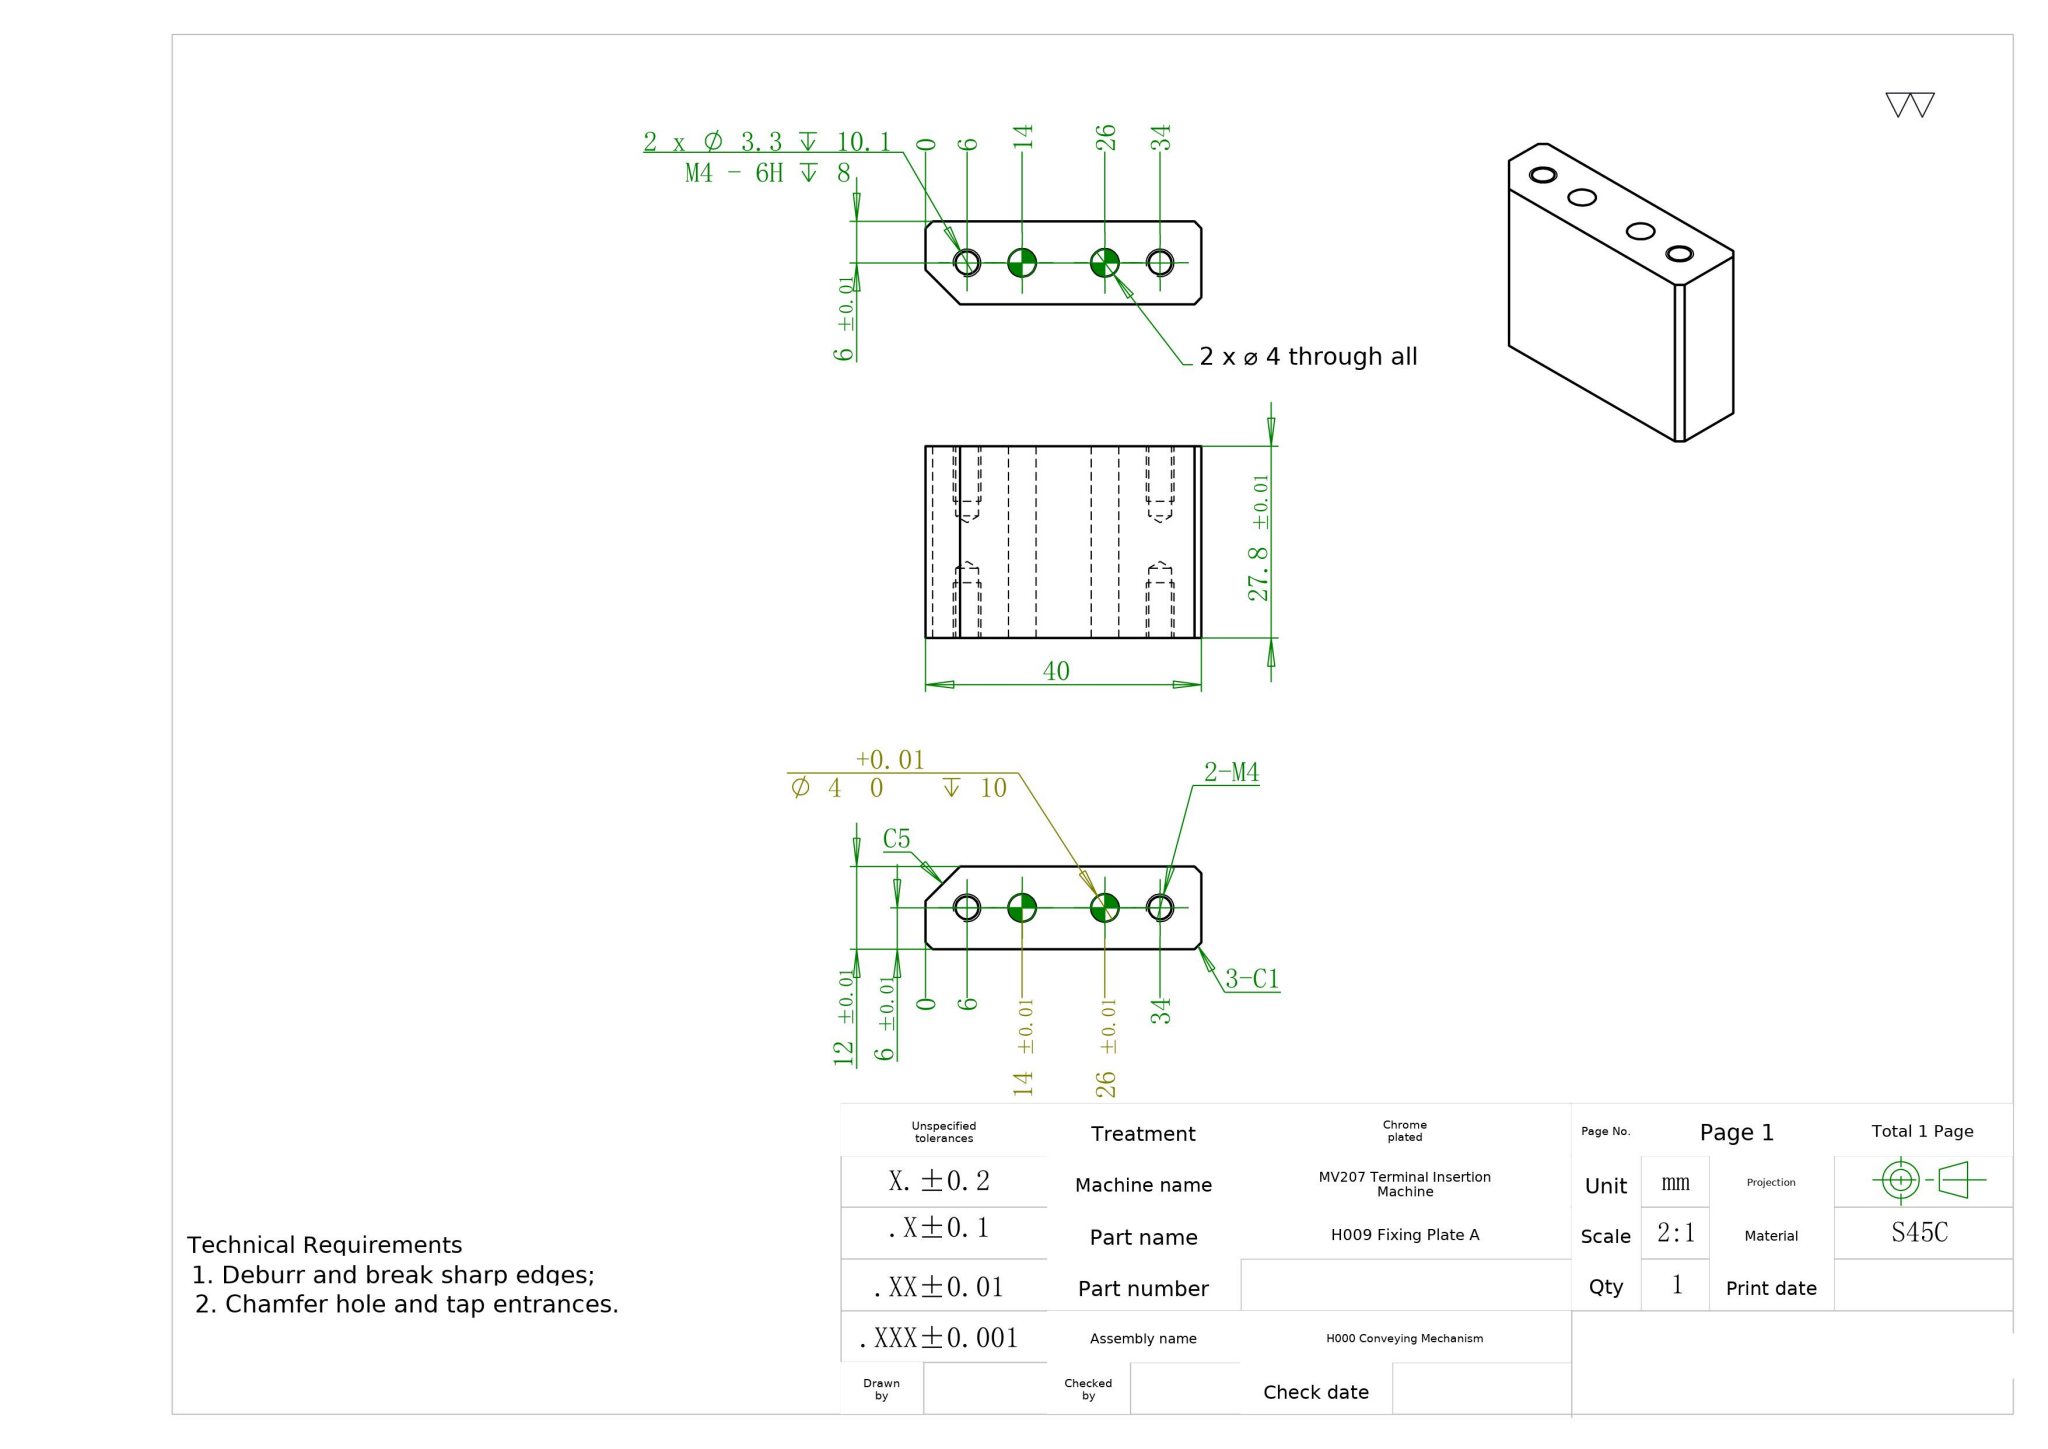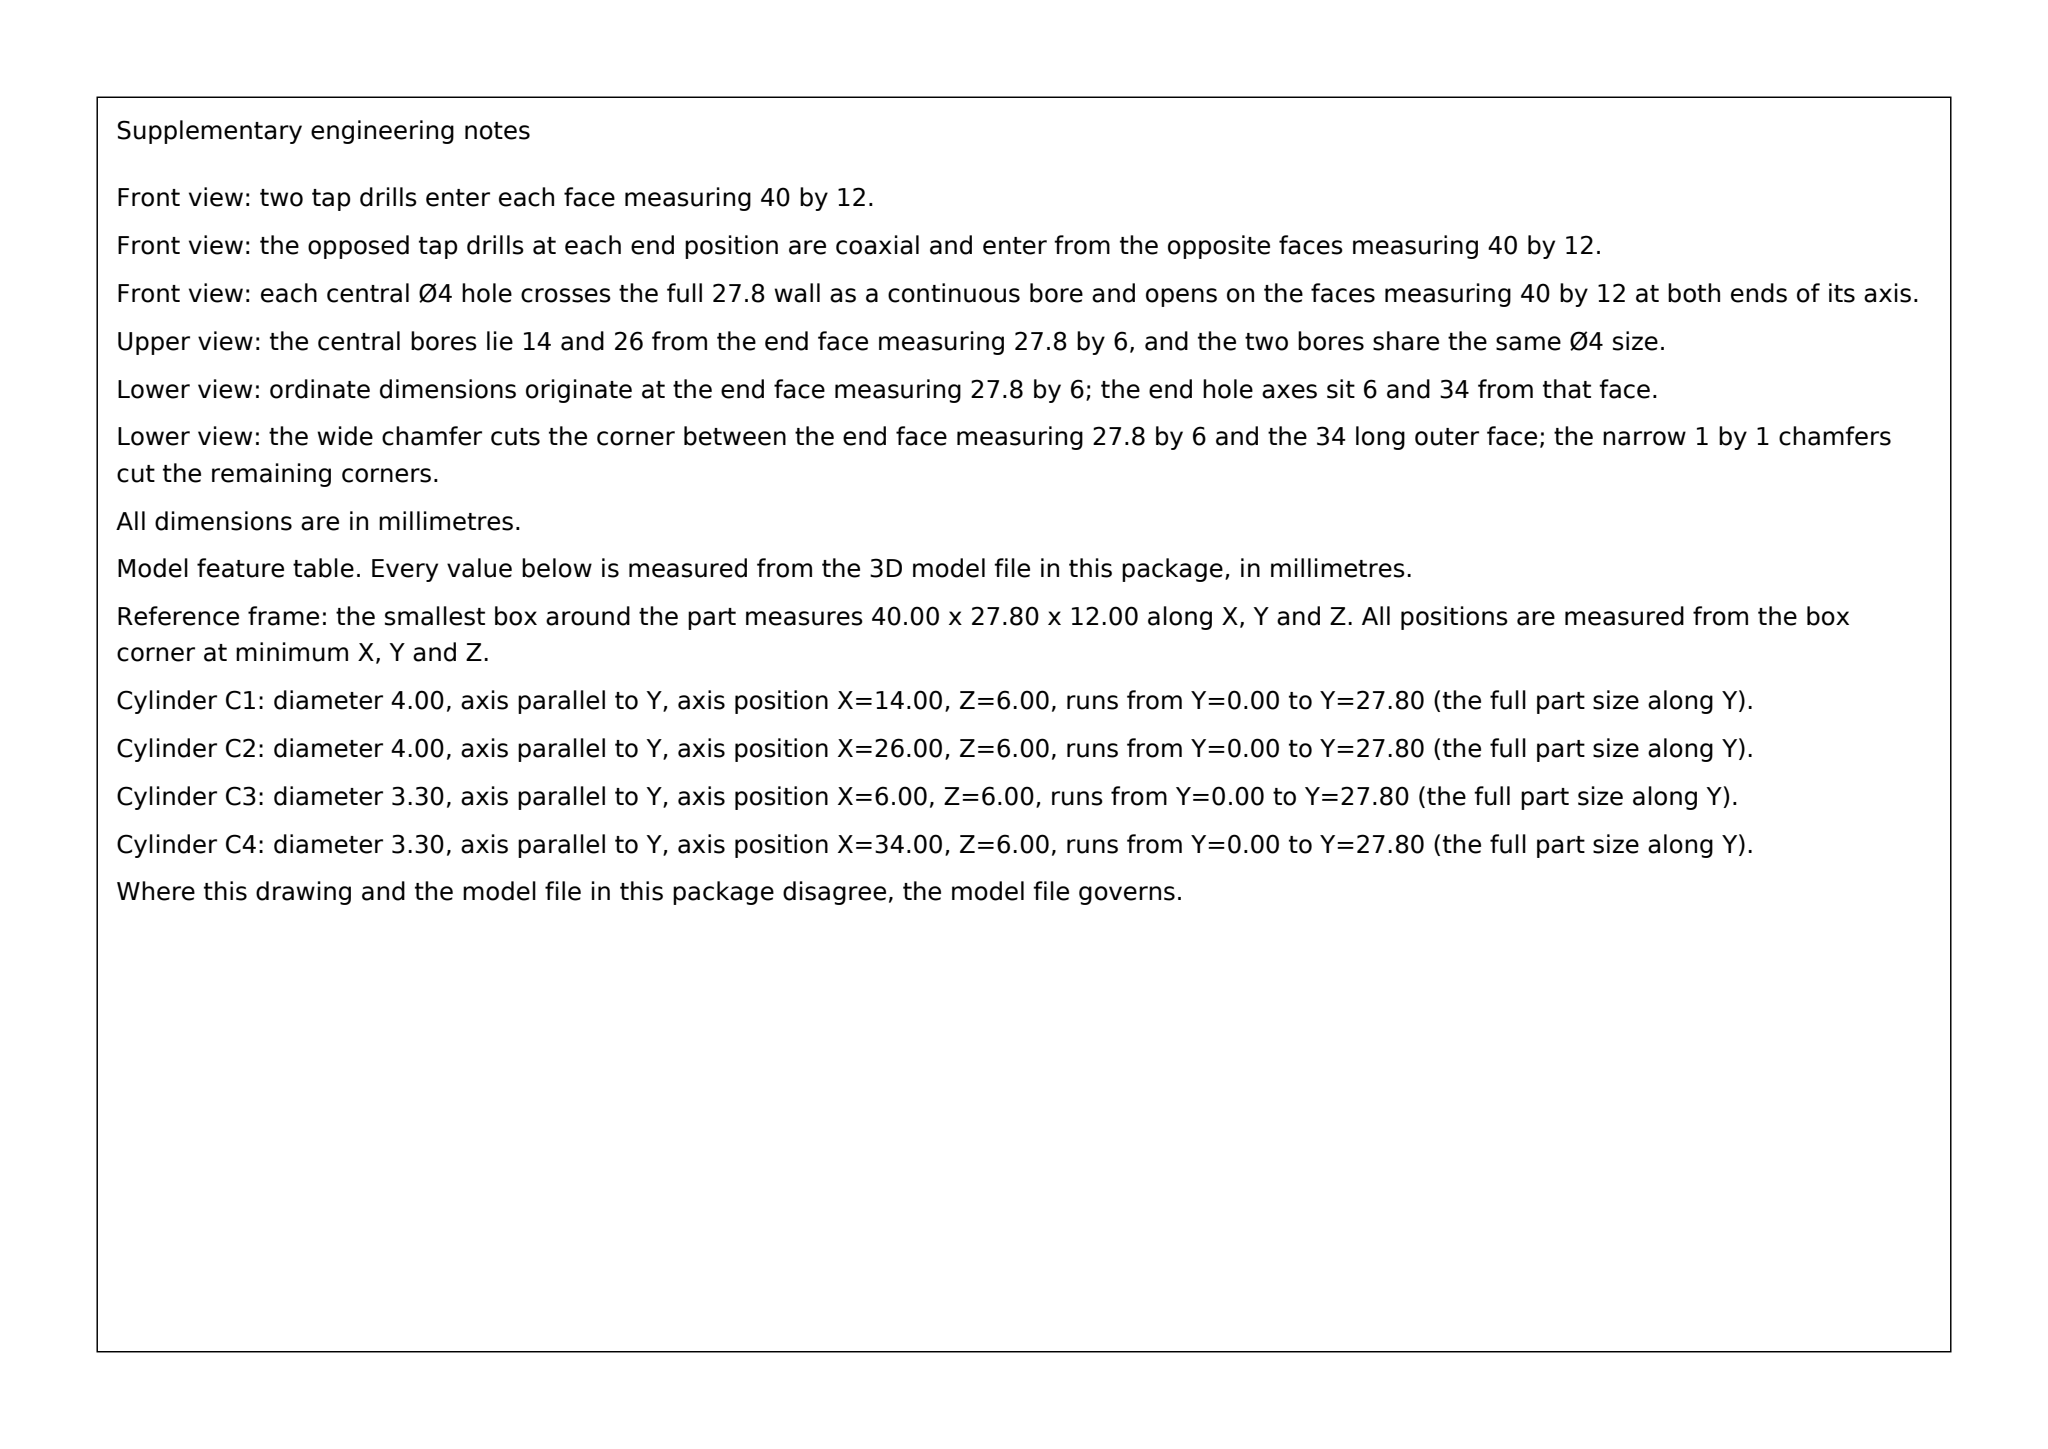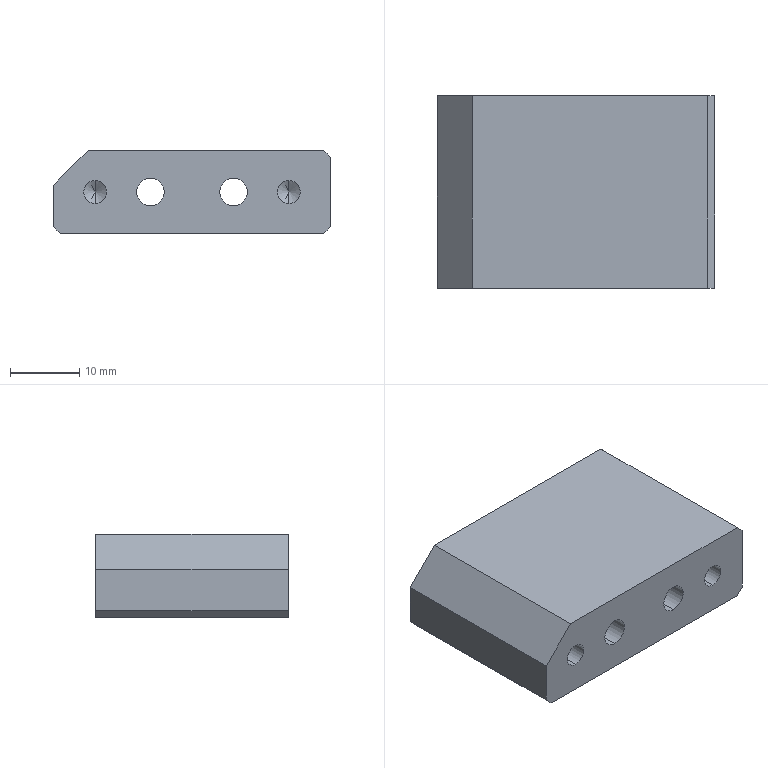Part | SolidWorks | mm | material S45C | 1 solid | 30 faces | box 40 x 27.8 x 12 mm | volume 11899 mm3 | cylinder 12 | plane 10 | cone 8 | commonest cylinder face diameters 3.3 x8 4 x4
Drawing notes:
2X Ø4 +0.01/0 THRU ALL = 27.8 DEEP (DISREGARD DP 10) | from the solid: Ø4 cylinders, axis Y, length 27.8 = full bbox Y (27.8) at x=14 & 26, z=6
TAPS: Ø3.3 DP 10.1 / M4-6H DP 8 FROM NEAREST 40X12 FACE | from the solid: Ø3.3 L=10.1 cyls (4 faces) + 8 cone faces @118°/Ø3.3 = 4 drill points, blind in 27.8 thk
4X M4-6H: 2 FROM TOP FACE, 2 FROM BOTTOM FACE, AT X=6 & 34, Z=6 | from the solid: Ø3.3 entries at [6,null,6] and [34,null,6], 4 cyl faces + 8 cone faces = 2 blind holes per location
DELETE C5: NO CHAMFER IN MODEL, CORNERS SQUARE 40 X 27.8 | from the solid: axis_planes only: x=0,40; y=0,27.8; z=0,12; no chamfer faces, fillet_radii=[]
DELETE 3-C1: NO C1 EDGES; ALL EDGES SHARP (BREAK EDGES ONLY) | from the solid: 6 planar faces form plain prism; no additional planar/conic edge faces present
PART IS PLAIN PRISM 40 X 27.8 X 12, NO CHAMFERS OR FILLETS | from the solid: bbox_xyz 40.0 x 27.8 x 12.0; 6 axis_planes; cones only 118 deg drill points on Ø3.3
build123d program:
from build123d import *

# Parameters (mm, degrees)
SKETCH1_W                    = 40
SKETCH1_H                    = 27.8
BOSS_EXTRUDE1_DEPTH          = 19.5
M4_TAPPED_HOLE2_D            = 3.3
M4_TAPPED_HOLE2_DEPTH        = 10.1
M4_TAPPED_HOLE2_TIP          = 0.9914
M4_TAPPED_HOLE1_D            = 3.3
M4_TAPPED_HOLE1_DEPTH        = 10.1
M4_TAPPED_HOLE1_TIP          = 0.9914
CHAMFER1_SIZE                = 5
F_4_0_4_DIAMETER_HOLE1_D     = 4
F_4_0_4_DIAMETER_HOLE2_D     = 4
F_4_0_4_DIAMETER_HOLE2_DEPTH = 10
F_4_0_4_DIAMETER_HOLE2_TIP   = 1.202
SKETCH15_W                   = 7.5
SKETCH15_H                   = 1.2
CUT_EXTRUDE1_DEPTH           = 47.62
SKETCH16_W                   = 40
SKETCH16_H                   = 25.4
CUT_EXTRUDE2_DEPTH           = 7.5
CHAMFER2_SIZE                = 1


with BuildPart() as part:
    # Sketch1 → Boss-Extrude1 (new body)
    with BuildSketch(Plane.XY):
        Rectangle(SKETCH1_W, SKETCH1_H)
    extrude(amount=BOSS_EXTRUDE1_DEPTH)

    # M4 Tapped Hole2
    with Locations(Plane(origin=(0, 13.9, 0), x_dir=(1, 0, 0), z_dir=(0, 1, 0))):
        with Locations((-14, -13.5), (14, -13.5)):
            Hole(M4_TAPPED_HOLE2_D / 2, depth=M4_TAPPED_HOLE2_DEPTH)
            with Locations((0, 0, -(M4_TAPPED_HOLE2_DEPTH + M4_TAPPED_HOLE2_TIP / 2))):  # 118° drill point
                Cone(0, M4_TAPPED_HOLE2_D / 2, M4_TAPPED_HOLE2_TIP, mode=Mode.SUBTRACT)

    # M4 Tapped Hole1
    with Locations(Plane(origin=(0, -13.9, 0), x_dir=(-1, 0, 0), z_dir=(0, -1, 0))):
        with Locations((14, -13.5), (-14, -13.5)):
            Hole(M4_TAPPED_HOLE1_D / 2, depth=M4_TAPPED_HOLE1_DEPTH)
            with Locations((0, 0, -(M4_TAPPED_HOLE1_DEPTH + M4_TAPPED_HOLE1_TIP / 2))):  # 118° drill point
                Cone(0, M4_TAPPED_HOLE1_D / 2, M4_TAPPED_HOLE1_TIP, mode=Mode.SUBTRACT)

    # Chamfer1
    chamfer1_edges = [part.edges().sort_by_distance(p)[0] for p in [
        (-20, 0, 19.5),
    ]]
    chamfer(chamfer1_edges, length=CHAMFER1_SIZE)

    # 4.0 _4_ Diameter Hole1 (through all)
    with Locations(Plane(origin=(0, 13.9, 0), x_dir=(1, 0, 0), z_dir=(0, 1, 0))):
        with Locations((-6, -13.5), (6, -13.5)):
            Hole(F_4_0_4_DIAMETER_HOLE1_D / 2)

    # 4.0 _4_ Diameter Hole2
    with Locations(Plane(origin=(0, -13.9, 0), x_dir=(-1, 0, 0), z_dir=(0, -1, 0))):
        with Locations((6, -13.5), (-6, -13.5)):
            Hole(F_4_0_4_DIAMETER_HOLE2_D / 2, depth=F_4_0_4_DIAMETER_HOLE2_DEPTH)
            with Locations((0, 0, -(F_4_0_4_DIAMETER_HOLE2_DEPTH + F_4_0_4_DIAMETER_HOLE2_TIP / 2))):  # 118° drill point
                Cone(0, F_4_0_4_DIAMETER_HOLE2_D / 2, F_4_0_4_DIAMETER_HOLE2_TIP, mode=Mode.SUBTRACT)

    # Sketch15 → Cut-Extrude1 (cut, through all)
    with BuildSketch(Plane(origin=(20, 0, 0), x_dir=(0, 0, -1), z_dir=(1, 0, 0))):
        with Locations((-3.75, -13.3)):
            Rectangle(SKETCH15_W, SKETCH15_H)
        with Locations((-3.75, 13.3)):
            Rectangle(SKETCH15_W, SKETCH15_H)
    extrude(amount=-CUT_EXTRUDE1_DEPTH, mode=Mode.SUBTRACT)

    # Sketch16 → Cut-Extrude2 (cut)
    with BuildSketch(Plane(origin=(0, 0, 0), x_dir=(-1, 0, 0), z_dir=(0, 0, -1))):
        Rectangle(SKETCH16_W, SKETCH16_H)
    extrude(amount=-CUT_EXTRUDE2_DEPTH, mode=Mode.SUBTRACT)

    # Chamfer2
    chamfer2_edges = [part.edges().sort_by_distance(p)[0] for p in [
        (20, 0, 19.5),
        (-20, 0, 7.5),
        (20, 0, 7.5),
    ]]
    chamfer(chamfer2_edges, length=CHAMFER2_SIZE)


solid = part.part
STEP:
#1=CARTESIAN_POINT('',(-6.,-13.9,11.5));
#2=VERTEX_POINT('',#1);
#3=CARTESIAN_POINT('',(-6.,-13.9,15.5));
#4=VERTEX_POINT('',#3);
#5=CARTESIAN_POINT('',(-6.,-13.9,13.5));
#6=DIRECTION('',(0.,1.,0.));
#7=DIRECTION('',(0.,0.,1.));
#8=AXIS2_PLACEMENT_3D('',#5,#6,#7);
#9=CIRCLE('',#8,2.);
#10=EDGE_CURVE('',#2,#4,#9,.T.);
#11=ORIENTED_EDGE('',*,*,#10,.F.);
#12=CARTESIAN_POINT('',(-6.,13.9,11.5));
#13=VERTEX_POINT('',#12);
#14=CARTESIAN_POINT('',(-6.,13.9,11.5));
#15=DIRECTION('',(0.,1.,0.));
#16=VECTOR('',#15,1000.);
#17=LINE('',#14,#16);
#18=EDGE_CURVE('',#2,#13,#17,.T.);
#19=ORIENTED_EDGE('',*,*,#18,.T.);
#20=CARTESIAN_POINT('',(-6.,13.9,15.5));
#21=VERTEX_POINT('',#20);
#22=CARTESIAN_POINT('',(-6.,13.9,13.5));
#23=DIRECTION('',(0.,1.,0.));
#24=DIRECTION('',(0.,0.,1.));
#25=AXIS2_PLACEMENT_3D('',#22,#23,#24);
#26=CIRCLE('',#25,2.);
#27=EDGE_CURVE('',#13,#21,#26,.T.);
#28=ORIENTED_EDGE('',*,*,#27,.T.);
#29=CARTESIAN_POINT('',(-6.,13.9,15.5));
#30=DIRECTION('',(0.,1.,0.));
#31=VECTOR('',#30,1000.);
#32=LINE('',#29,#31);
#33=EDGE_CURVE('',#4,#21,#32,.T.);
#34=ORIENTED_EDGE('',*,*,#33,.F.);
#35=EDGE_LOOP('',(#11,#19,#28,#34));
#36=FACE_OUTER_BOUND('',#35,.T.);
#37=CARTESIAN_POINT('',(-6.,13.9,13.5));
#38=DIRECTION('',(0.,1.,0.));
#39=DIRECTION('',(0.,0.,1.));
#40=AXIS2_PLACEMENT_3D('',#37,#38,#39);
#41=CYLINDRICAL_SURFACE('',#40,2.);
#42=ADVANCED_FACE('',(#36),#41,.F.);
#43=CARTESIAN_POINT('',(6.,-13.9,11.5));
#44=VERTEX_POINT('',#43);
#45=CARTESIAN_POINT('',(6.,-13.9,15.5));
#46=VERTEX_POINT('',#45);
#47=CARTESIAN_POINT('',(6.,-13.9,13.5));
#48=DIRECTION('',(0.,1.,0.));
#49=DIRECTION('',(0.,0.,1.));
#50=AXIS2_PLACEMENT_3D('',#47,#48,#49);
#51=CIRCLE('',#50,2.);
#52=EDGE_CURVE('',#44,#46,#51,.T.);
#53=ORIENTED_EDGE('',*,*,#52,.F.);
#54=CARTESIAN_POINT('',(6.,13.9,11.5));
#55=VERTEX_POINT('',#54);
#56=CARTESIAN_POINT('',(6.,13.9,11.5));
#57=DIRECTION('',(0.,1.,0.));
#58=VECTOR('',#57,1000.);
#59=LINE('',#56,#58);
#60=EDGE_CURVE('',#44,#55,#59,.T.);
#61=ORIENTED_EDGE('',*,*,#60,.T.);
#62=CARTESIAN_POINT('',(6.,13.9,15.5));
#63=VERTEX_POINT('',#62);
#64=CARTESIAN_POINT('',(6.,13.9,13.5));
#65=DIRECTION('',(0.,1.,0.));
#66=DIRECTION('',(0.,0.,1.));
#67=AXIS2_PLACEMENT_3D('',#64,#65,#66);
#68=CIRCLE('',#67,2.);
#69=EDGE_CURVE('',#55,#63,#68,.T.);
#70=ORIENTED_EDGE('',*,*,#69,.T.);
#71=CARTESIAN_POINT('',(6.,13.9,15.5));
#72=DIRECTION('',(0.,1.,0.));
#73=VECTOR('',#72,1000.);
#74=LINE('',#71,#73);
#75=EDGE_CURVE('',#46,#63,#74,.T.);
#76=ORIENTED_EDGE('',*,*,#75,.F.);
#77=EDGE_LOOP('',(#53,#61,#70,#76));
#78=FACE_OUTER_BOUND('',#77,.T.);
#79=CARTESIAN_POINT('',(6.,13.9,13.5));
#80=DIRECTION('',(0.,1.,0.));
#81=DIRECTION('',(0.,0.,1.));
#82=AXIS2_PLACEMENT_3D('',#79,#80,#81);
#83=CYLINDRICAL_SURFACE('',#82,2.);
#84=ADVANCED_FACE('',(#78),#83,.F.);
#85=CARTESIAN_POINT('',(-14.,-3.8,15.15));
#86=VERTEX_POINT('',#85);
#87=CARTESIAN_POINT('',(-14.,-3.8,11.85));
#88=VERTEX_POINT('',#87);
#89=CARTESIAN_POINT('',(-14.,-3.8,13.5));
#90=DIRECTION('',(0.,-1.,0.));
#91=DIRECTION('',(0.,0.,-1.));
#92=AXIS2_PLACEMENT_3D('',#89,#90,#91);
#93=CIRCLE('',#92,1.65);
#94=EDGE_CURVE('',#86,#88,#93,.T.);
#95=ORIENTED_EDGE('',*,*,#94,.F.);
#96=CARTESIAN_POINT('',(-14.,-13.9,15.15));
#97=VERTEX_POINT('',#96);
#98=CARTESIAN_POINT('',(-14.,-13.9,15.15));
#99=DIRECTION('',(0.,-1.,0.));
#100=VECTOR('',#99,1000.);
#101=LINE('',#98,#100);
#102=EDGE_CURVE('',#86,#97,#101,.T.);
#103=ORIENTED_EDGE('',*,*,#102,.T.);
#104=CARTESIAN_POINT('',(-14.,-13.9,11.85));
#105=VERTEX_POINT('',#104);
#106=CARTESIAN_POINT('',(-14.,-13.9,13.5));
#107=DIRECTION('',(0.,-1.,0.));
#108=DIRECTION('',(0.,0.,-1.));
#109=AXIS2_PLACEMENT_3D('',#106,#107,#108);
#110=CIRCLE('',#109,1.65);
#111=EDGE_CURVE('',#97,#105,#110,.T.);
#112=ORIENTED_EDGE('',*,*,#111,.T.);
#113=CARTESIAN_POINT('',(-14.,-13.9,11.85));
#114=DIRECTION('',(0.,-1.,0.));
#115=VECTOR('',#114,1000.);
#116=LINE('',#113,#115);
#117=EDGE_CURVE('',#88,#105,#116,.T.);
#118=ORIENTED_EDGE('',*,*,#117,.F.);
#119=EDGE_LOOP('',(#95,#103,#112,#118));
#120=FACE_OUTER_BOUND('',#119,.T.);
#121=CARTESIAN_POINT('',(-14.,-13.9,13.5));
#122=DIRECTION('',(0.,-1.,0.));
#123=DIRECTION('',(0.,0.,-1.));
#124=AXIS2_PLACEMENT_3D('',#121,#122,#123);
#125=CYLINDRICAL_SURFACE('',#124,1.65);
#126=ADVANCED_FACE('',(#120),#125,.F.);
#127=CARTESIAN_POINT('',(-14.,-2.809,13.5));
#128=VERTEX_POINT('',#127);
#129=CARTESIAN_POINT('',(-14.,-3.8,11.85));
#130=DIRECTION('',(0.,-0.515,-0.8572));
#131=VECTOR('',#130,1000.);
#132=LINE('',#129,#131);
#133=EDGE_CURVE('',#128,#88,#132,.T.);
#134=ORIENTED_EDGE('',*,*,#133,.F.);
#135=CARTESIAN_POINT('',(-14.,-3.8,15.15));
#136=DIRECTION('',(0.,-0.515,0.8572));
#137=VECTOR('',#136,1000.);
#138=LINE('',#135,#137);
#139=EDGE_CURVE('',#128,#86,#138,.T.);
#140=ORIENTED_EDGE('',*,*,#139,.T.);
#141=ORIENTED_EDGE('',*,*,#94,.T.);
#142=EDGE_LOOP('',(#134,#140,#141));
#143=FACE_OUTER_BOUND('',#142,.T.);
#144=CARTESIAN_POINT('',(-14.,-3.8,13.5));
#145=DIRECTION('',(0.,-1.,0.));
#146=DIRECTION('',(0.,0.,-1.));
#147=AXIS2_PLACEMENT_3D('',#144,#145,#146);
#148=CONICAL_SURFACE('',#147,1.65,1.03);
#149=ADVANCED_FACE('',(#143),#148,.F.);
#150=CARTESIAN_POINT('',(14.,-3.8,15.15));
#151=VERTEX_POINT('',#150);
#152=CARTESIAN_POINT('',(14.,-3.8,11.85));
#153=VERTEX_POINT('',#152);
#154=CARTESIAN_POINT('',(14.,-3.8,13.5));
#155=DIRECTION('',(0.,-1.,0.));
#156=DIRECTION('',(0.,0.,-1.));
#157=AXIS2_PLACEMENT_3D('',#154,#155,#156);
#158=CIRCLE('',#157,1.65);
#159=EDGE_CURVE('',#151,#153,#158,.T.);
#160=ORIENTED_EDGE('',*,*,#159,.F.);
#161=CARTESIAN_POINT('',(14.,-13.9,15.15));
#162=VERTEX_POINT('',#161);
#163=CARTESIAN_POINT('',(14.,-13.9,15.15));
#164=DIRECTION('',(0.,-1.,0.));
#165=VECTOR('',#164,1000.);
#166=LINE('',#163,#165);
#167=EDGE_CURVE('',#151,#162,#166,.T.);
#168=ORIENTED_EDGE('',*,*,#167,.T.);
#169=CARTESIAN_POINT('',(14.,-13.9,11.85));
#170=VERTEX_POINT('',#169);
#171=CARTESIAN_POINT('',(14.,-13.9,13.5));
#172=DIRECTION('',(0.,-1.,0.));
#173=DIRECTION('',(0.,0.,-1.));
#174=AXIS2_PLACEMENT_3D('',#171,#172,#173);
#175=CIRCLE('',#174,1.65);
#176=EDGE_CURVE('',#162,#170,#175,.T.);
#177=ORIENTED_EDGE('',*,*,#176,.T.);
#178=CARTESIAN_POINT('',(14.,-13.9,11.85));
#179=DIRECTION('',(0.,-1.,0.));
#180=VECTOR('',#179,1000.);
#181=LINE('',#178,#180);
#182=EDGE_CURVE('',#153,#170,#181,.T.);
#183=ORIENTED_EDGE('',*,*,#182,.F.);
#184=EDGE_LOOP('',(#160,#168,#177,#183));
#185=FACE_OUTER_BOUND('',#184,.T.);
#186=CARTESIAN_POINT('',(14.,-13.9,13.5));
#187=DIRECTION('',(0.,-1.,0.));
#188=DIRECTION('',(0.,0.,-1.));
#189=AXIS2_PLACEMENT_3D('',#186,#187,#188);
#190=CYLINDRICAL_SURFACE('',#189,1.65);
#191=ADVANCED_FACE('',(#185),#190,.F.);
#192=CARTESIAN_POINT('',(14.,-2.809,13.5));
#193=VERTEX_POINT('',#192);
#194=CARTESIAN_POINT('',(14.,-3.8,11.85));
#195=DIRECTION('',(0.,-0.515,-0.8572));
#196=VECTOR('',#195,1000.);
#197=LINE('',#194,#196);
#198=EDGE_CURVE('',#193,#153,#197,.T.);
#199=ORIENTED_EDGE('',*,*,#198,.F.);
#200=CARTESIAN_POINT('',(14.,-3.8,15.15));
#201=DIRECTION('',(0.,-0.515,0.8572));
#202=VECTOR('',#201,1000.);
#203=LINE('',#200,#202);
#204=EDGE_CURVE('',#193,#151,#203,.T.);
#205=ORIENTED_EDGE('',*,*,#204,.T.);
#206=ORIENTED_EDGE('',*,*,#159,.T.);
#207=EDGE_LOOP('',(#199,#205,#206));
#208=FACE_OUTER_BOUND('',#207,.T.);
#209=CARTESIAN_POINT('',(14.,-3.8,13.5));
#210=DIRECTION('',(0.,-1.,0.));
#211=DIRECTION('',(0.,0.,-1.));
#212=AXIS2_PLACEMENT_3D('',#209,#210,#211);
#213=CONICAL_SURFACE('',#212,1.65,1.03);
#214=ADVANCED_FACE('',(#208),#213,.F.);
#215=CARTESIAN_POINT('',(-14.,3.8,11.85));
#216=VERTEX_POINT('',#215);
#217=CARTESIAN_POINT('',(-14.,3.8,15.15));
#218=VERTEX_POINT('',#217);
#219=CARTESIAN_POINT('',(-14.,3.8,13.5));
#220=DIRECTION('',(0.,1.,0.));
#221=DIRECTION('',(0.,0.,1.));
#222=AXIS2_PLACEMENT_3D('',#219,#220,#221);
#223=CIRCLE('',#222,1.65);
#224=EDGE_CURVE('',#216,#218,#223,.T.);
#225=ORIENTED_EDGE('',*,*,#224,.F.);
#226=CARTESIAN_POINT('',(-14.,13.9,11.85));
#227=VERTEX_POINT('',#226);
#228=CARTESIAN_POINT('',(-14.,13.9,11.85));
#229=DIRECTION('',(0.,1.,0.));
#230=VECTOR('',#229,1000.);
#231=LINE('',#228,#230);
#232=EDGE_CURVE('',#216,#227,#231,.T.);
#233=ORIENTED_EDGE('',*,*,#232,.T.);
#234=CARTESIAN_POINT('',(-14.,13.9,15.15));
#235=VERTEX_POINT('',#234);
#236=CARTESIAN_POINT('',(-14.,13.9,13.5));
#237=DIRECTION('',(0.,1.,0.));
#238=DIRECTION('',(0.,0.,1.));
#239=AXIS2_PLACEMENT_3D('',#236,#237,#238);
#240=CIRCLE('',#239,1.65);
#241=EDGE_CURVE('',#227,#235,#240,.T.);
#242=ORIENTED_EDGE('',*,*,#241,.T.);
#243=CARTESIAN_POINT('',(-14.,13.9,15.15));
#244=DIRECTION('',(0.,1.,0.));
#245=VECTOR('',#244,1000.);
#246=LINE('',#243,#245);
#247=EDGE_CURVE('',#218,#235,#246,.T.);
#248=ORIENTED_EDGE('',*,*,#247,.F.);
#249=EDGE_LOOP('',(#225,#233,#242,#248));
#250=FACE_OUTER_BOUND('',#249,.T.);
#251=CARTESIAN_POINT('',(-14.,13.9,13.5));
#252=DIRECTION('',(0.,1.,0.));
#253=DIRECTION('',(0.,0.,1.));
#254=AXIS2_PLACEMENT_3D('',#251,#252,#253);
#255=CYLINDRICAL_SURFACE('',#254,1.65);
#256=ADVANCED_FACE('',(#250),#255,.F.);
#257=CARTESIAN_POINT('',(-14.,2.809,13.5));
#258=VERTEX_POINT('',#257);
#259=CARTESIAN_POINT('',(-14.,3.8,15.15));
#260=DIRECTION('',(0.,0.515,0.8572));
#261=VECTOR('',#260,1000.);
#262=LINE('',#259,#261);
#263=EDGE_CURVE('',#258,#218,#262,.T.);
#264=ORIENTED_EDGE('',*,*,#263,.F.);
#265=CARTESIAN_POINT('',(-14.,3.8,11.85));
#266=DIRECTION('',(0.,0.515,-0.8572));
#267=VECTOR('',#266,1000.);
#268=LINE('',#265,#267);
#269=EDGE_CURVE('',#258,#216,#268,.T.);
#270=ORIENTED_EDGE('',*,*,#269,.T.);
#271=ORIENTED_EDGE('',*,*,#224,.T.);
#272=EDGE_LOOP('',(#264,#270,#271));
#273=FACE_OUTER_BOUND('',#272,.T.);
#274=CARTESIAN_POINT('',(-14.,3.8,13.5));
#275=DIRECTION('',(0.,1.,0.));
#276=DIRECTION('',(0.,0.,1.));
#277=AXIS2_PLACEMENT_3D('',#274,#275,#276);
#278=CONICAL_SURFACE('',#277,1.65,1.03);
#279=ADVANCED_FACE('',(#273),#278,.F.);
#280=CARTESIAN_POINT('',(14.,3.8,11.85));
#281=VERTEX_POINT('',#280);
#282=CARTESIAN_POINT('',(14.,3.8,15.15));
#283=VERTEX_POINT('',#282);
#284=CARTESIAN_POINT('',(14.,3.8,13.5));
#285=DIRECTION('',(0.,1.,0.));
#286=DIRECTION('',(0.,0.,1.));
#287=AXIS2_PLACEMENT_3D('',#284,#285,#286);
#288=CIRCLE('',#287,1.65);
#289=EDGE_CURVE('',#281,#283,#288,.T.);
#290=ORIENTED_EDGE('',*,*,#289,.F.);
#291=CARTESIAN_POINT('',(14.,13.9,11.85));
#292=VERTEX_POINT('',#291);
#293=CARTESIAN_POINT('',(14.,13.9,11.85));
#294=DIRECTION('',(0.,1.,0.));
#295=VECTOR('',#294,1000.);
#296=LINE('',#293,#295);
#297=EDGE_CURVE('',#281,#292,#296,.T.);
#298=ORIENTED_EDGE('',*,*,#297,.T.);
#299=CARTESIAN_POINT('',(14.,13.9,15.15));
#300=VERTEX_POINT('',#299);
#301=CARTESIAN_POINT('',(14.,13.9,13.5));
#302=DIRECTION('',(0.,1.,0.));
#303=DIRECTION('',(0.,0.,1.));
#304=AXIS2_PLACEMENT_3D('',#301,#302,#303);
#305=CIRCLE('',#304,1.65);
#306=EDGE_CURVE('',#292,#300,#305,.T.);
#307=ORIENTED_EDGE('',*,*,#306,.T.);
#308=CARTESIAN_POINT('',(14.,13.9,15.15));
#309=DIRECTION('',(0.,1.,0.));
#310=VECTOR('',#309,1000.);
#311=LINE('',#308,#310);
#312=EDGE_CURVE('',#283,#300,#311,.T.);
#313=ORIENTED_EDGE('',*,*,#312,.F.);
#314=EDGE_LOOP('',(#290,#298,#307,#313));
#315=FACE_OUTER_BOUND('',#314,.T.);
#316=CARTESIAN_POINT('',(14.,13.9,13.5));
#317=DIRECTION('',(0.,1.,0.));
#318=DIRECTION('',(0.,0.,1.));
#319=AXIS2_PLACEMENT_3D('',#316,#317,#318);
#320=CYLINDRICAL_SURFACE('',#319,1.65);
#321=ADVANCED_FACE('',(#315),#320,.F.);
#322=CARTESIAN_POINT('',(14.,2.809,13.5));
#323=VERTEX_POINT('',#322);
#324=CARTESIAN_POINT('',(14.,3.8,15.15));
#325=DIRECTION('',(0.,0.515,0.8572));
#326=VECTOR('',#325,1000.);
#327=LINE('',#324,#326);
#328=EDGE_CURVE('',#323,#283,#327,.T.);
#329=ORIENTED_EDGE('',*,*,#328,.F.);
#330=CARTESIAN_POINT('',(14.,3.8,11.85));
#331=DIRECTION('',(0.,0.515,-0.8572));
#332=VECTOR('',#331,1000.);
#333=LINE('',#330,#332);
#334=EDGE_CURVE('',#323,#281,#333,.T.);
#335=ORIENTED_EDGE('',*,*,#334,.T.);
#336=ORIENTED_EDGE('',*,*,#289,.T.);
#337=EDGE_LOOP('',(#329,#335,#336));
#338=FACE_OUTER_BOUND('',#337,.T.);
#339=CARTESIAN_POINT('',(14.,3.8,13.5));
#340=DIRECTION('',(0.,1.,0.));
#341=DIRECTION('',(0.,0.,1.));
#342=AXIS2_PLACEMENT_3D('',#339,#340,#341);
#343=CONICAL_SURFACE('',#342,1.65,1.03);
#344=ADVANCED_FACE('',(#338),#343,.F.);
#345=CARTESIAN_POINT('',(20.,13.9,18.5));
#346=VERTEX_POINT('',#345);
#347=CARTESIAN_POINT('',(20.,13.9,8.5));
#348=VERTEX_POINT('',#347);
#349=CARTESIAN_POINT('',(20.,13.9,19.5));
#350=DIRECTION('',(0.,0.,-1.));
#351=VECTOR('',#350,1000.);
#352=LINE('',#349,#351);
#353=EDGE_CURVE('',#346,#348,#352,.T.);
#354=ORIENTED_EDGE('',*,*,#353,.F.);
#355=CARTESIAN_POINT('',(20.,-13.9,18.5));
#356=VERTEX_POINT('',#355);
#357=CARTESIAN_POINT('',(20.,-13.9,18.5));
#358=DIRECTION('',(0.,-1.,0.));
#359=VECTOR('',#358,1000.);
#360=LINE('',#357,#359);
#361=EDGE_CURVE('',#346,#356,#360,.T.);
#362=ORIENTED_EDGE('',*,*,#361,.T.);
#363=CARTESIAN_POINT('',(20.,-13.9,8.5));
#364=VERTEX_POINT('',#363);
#365=CARTESIAN_POINT('',(20.,-13.9,19.5));
#366=DIRECTION('',(0.,0.,-1.));
#367=VECTOR('',#366,1000.);
#368=LINE('',#365,#367);
#369=EDGE_CURVE('',#356,#364,#368,.T.);
#370=ORIENTED_EDGE('',*,*,#369,.T.);
#371=CARTESIAN_POINT('',(20.,13.9,8.5));
#372=DIRECTION('',(0.,1.,0.));
#373=VECTOR('',#372,1000.);
#374=LINE('',#371,#373);
#375=EDGE_CURVE('',#364,#348,#374,.T.);
#376=ORIENTED_EDGE('',*,*,#375,.T.);
#377=EDGE_LOOP('',(#354,#362,#370,#376));
#378=FACE_OUTER_BOUND('',#377,.T.);
#379=CARTESIAN_POINT('',(20.,13.9,19.5));
#380=DIRECTION('',(-1.,0.,0.));
#381=DIRECTION('',(0.,0.,1.));
#382=AXIS2_PLACEMENT_3D('',#379,#380,#381);
#383=PLANE('',#382);
#384=ADVANCED_FACE('',(#378),#383,.F.);
#385=CARTESIAN_POINT('',(-6.,13.9,13.5));
#386=DIRECTION('',(0.,1.,0.));
#387=DIRECTION('',(0.,0.,1.));
#388=AXIS2_PLACEMENT_3D('',#385,#386,#387);
#389=CIRCLE('',#388,2.);
#390=EDGE_CURVE('',#21,#13,#389,.T.);
#391=ORIENTED_EDGE('',*,*,#390,.F.);
#392=ORIENTED_EDGE('',*,*,#27,.F.);
#393=EDGE_LOOP('',(#391,#392));
#394=FACE_BOUND('',#393,.T.);
#395=CARTESIAN_POINT('',(6.,13.9,13.5));
#396=DIRECTION('',(0.,1.,0.));
#397=DIRECTION('',(0.,0.,1.));
#398=AXIS2_PLACEMENT_3D('',#395,#396,#397);
#399=CIRCLE('',#398,2.);
#400=EDGE_CURVE('',#63,#55,#399,.T.);
#401=ORIENTED_EDGE('',*,*,#400,.F.);
#402=ORIENTED_EDGE('',*,*,#69,.F.);
#403=EDGE_LOOP('',(#401,#402));
#404=FACE_BOUND('',#403,.T.);
#405=CARTESIAN_POINT('',(-14.,13.9,13.5));
#406=DIRECTION('',(0.,1.,0.));
#407=DIRECTION('',(0.,0.,1.));
#408=AXIS2_PLACEMENT_3D('',#405,#406,#407);
#409=CIRCLE('',#408,1.65);
#410=EDGE_CURVE('',#235,#227,#409,.T.);
#411=ORIENTED_EDGE('',*,*,#410,.F.);
#412=ORIENTED_EDGE('',*,*,#241,.F.);
#413=EDGE_LOOP('',(#411,#412));
#414=FACE_BOUND('',#413,.T.);
#415=CARTESIAN_POINT('',(14.,13.9,13.5));
#416=DIRECTION('',(0.,1.,0.));
#417=DIRECTION('',(0.,0.,1.));
#418=AXIS2_PLACEMENT_3D('',#415,#416,#417);
#419=CIRCLE('',#418,1.65);
#420=EDGE_CURVE('',#300,#292,#419,.T.);
#421=ORIENTED_EDGE('',*,*,#420,.F.);
#422=ORIENTED_EDGE('',*,*,#306,.F.);
#423=EDGE_LOOP('',(#421,#422));
#424=FACE_BOUND('',#423,.T.);
#425=CARTESIAN_POINT('',(19.,13.9,19.5));
#426=VERTEX_POINT('',#425);
#427=CARTESIAN_POINT('',(-15.,13.9,19.5));
#428=VERTEX_POINT('',#427);
#429=CARTESIAN_POINT('',(-20.,13.9,19.5));
#430=DIRECTION('',(-1.,0.,0.));
#431=VECTOR('',#430,1000.);
#432=LINE('',#429,#431);
#433=EDGE_CURVE('',#426,#428,#432,.T.);
#434=ORIENTED_EDGE('',*,*,#433,.F.);
#435=CARTESIAN_POINT('',(19.,13.9,19.5));
#436=DIRECTION('',(0.7071,0.,-0.7071));
#437=VECTOR('',#436,1000.);
#438=LINE('',#435,#437);
#439=EDGE_CURVE('',#426,#346,#438,.T.);
#440=ORIENTED_EDGE('',*,*,#439,.T.);
#441=ORIENTED_EDGE('',*,*,#353,.T.);
#442=CARTESIAN_POINT('',(19.,13.9,7.5));
#443=VERTEX_POINT('',#442);
#444=CARTESIAN_POINT('',(19.,13.9,7.5));
#445=DIRECTION('',(-0.7071,0.,-0.7071));
#446=VECTOR('',#445,1000.);
#447=LINE('',#444,#446);
#448=EDGE_CURVE('',#348,#443,#447,.T.);
#449=ORIENTED_EDGE('',*,*,#448,.T.);
#450=CARTESIAN_POINT('',(-19.,13.9,7.5));
#451=VERTEX_POINT('',#450);
#452=CARTESIAN_POINT('',(-20.,13.9,7.5));
#453=DIRECTION('',(1.,0.,0.));
#454=VECTOR('',#453,1000.);
#455=LINE('',#452,#454);
#456=EDGE_CURVE('',#451,#443,#455,.T.);
#457=ORIENTED_EDGE('',*,*,#456,.F.);
#458=CARTESIAN_POINT('',(-20.,13.9,8.5));
#459=VERTEX_POINT('',#458);
#460=CARTESIAN_POINT('',(-20.,13.9,8.5));
#461=DIRECTION('',(-0.7071,0.,0.7071));
#462=VECTOR('',#461,1000.);
#463=LINE('',#460,#462);
#464=EDGE_CURVE('',#451,#459,#463,.T.);
#465=ORIENTED_EDGE('',*,*,#464,.T.);
#466=CARTESIAN_POINT('',(-20.,13.9,14.5));
#467=VERTEX_POINT('',#466);
#468=CARTESIAN_POINT('',(-20.,13.9,19.5));
#469=DIRECTION('',(0.,0.,-1.));
#470=VECTOR('',#469,1000.);
#471=LINE('',#468,#470);
#472=EDGE_CURVE('',#467,#459,#471,.T.);
#473=ORIENTED_EDGE('',*,*,#472,.F.);
#474=CARTESIAN_POINT('',(-15.,13.9,19.5));
#475=DIRECTION('',(0.7071,0.,0.7071));
#476=VECTOR('',#475,1000.);
#477=LINE('',#474,#476);
#478=EDGE_CURVE('',#467,#428,#477,.T.);
#479=ORIENTED_EDGE('',*,*,#478,.T.);
#480=EDGE_LOOP('',(#434,#440,#441,#449,#457,#465,#473,#479));
#481=FACE_OUTER_BOUND('',#480,.T.);
#482=CARTESIAN_POINT('',(-20.,13.9,19.5));
#483=DIRECTION('',(0.,-1.,0.));
#484=DIRECTION('',(0.,0.,-1.));
#485=AXIS2_PLACEMENT_3D('',#482,#483,#484);
#486=PLANE('',#485);
#487=ADVANCED_FACE('',(#394,#404,#414,#424,#481),#486,.F.);
#488=ORIENTED_EDGE('',*,*,#472,.T.);
#489=CARTESIAN_POINT('',(-20.,-13.9,8.5));
#490=VERTEX_POINT('',#489);
#491=CARTESIAN_POINT('',(-20.,13.9,8.5));
#492=DIRECTION('',(0.,-1.,0.));
#493=VECTOR('',#492,1000.);
#494=LINE('',#491,#493);
#495=EDGE_CURVE('',#459,#490,#494,.T.);
#496=ORIENTED_EDGE('',*,*,#495,.T.);
#497=CARTESIAN_POINT('',(-20.,-13.9,14.5));
#498=VERTEX_POINT('',#497);
#499=CARTESIAN_POINT('',(-20.,-13.9,19.5));
#500=DIRECTION('',(0.,0.,-1.));
#501=VECTOR('',#500,1000.);
#502=LINE('',#499,#501);
#503=EDGE_CURVE('',#498,#490,#502,.T.);
#504=ORIENTED_EDGE('',*,*,#503,.F.);
#505=CARTESIAN_POINT('',(-20.,13.9,14.5));
#506=DIRECTION('',(0.,1.,0.));
#507=VECTOR('',#506,1000.);
#508=LINE('',#505,#507);
#509=EDGE_CURVE('',#498,#467,#508,.T.);
#510=ORIENTED_EDGE('',*,*,#509,.T.);
#511=EDGE_LOOP('',(#488,#496,#504,#510));
#512=FACE_OUTER_BOUND('',#511,.T.);
#513=CARTESIAN_POINT('',(-20.,13.9,19.5));
#514=DIRECTION('',(1.,0.,0.));
#515=DIRECTION('',(0.,0.,-1.));
#516=AXIS2_PLACEMENT_3D('',#513,#514,#515);
#517=PLANE('',#516);
#518=ADVANCED_FACE('',(#512),#517,.F.);
#519=CARTESIAN_POINT('',(-6.,-13.9,13.5));
#520=DIRECTION('',(0.,1.,0.));
#521=DIRECTION('',(0.,0.,1.));
#522=AXIS2_PLACEMENT_3D('',#519,#520,#521);
#523=CIRCLE('',#522,2.);
#524=EDGE_CURVE('',#4,#2,#523,.T.);
#525=ORIENTED_EDGE('',*,*,#524,.T.);
#526=ORIENTED_EDGE('',*,*,#10,.T.);
#527=EDGE_LOOP('',(#525,#526));
#528=FACE_BOUND('',#527,.T.);
#529=CARTESIAN_POINT('',(6.,-13.9,13.5));
#530=DIRECTION('',(0.,1.,0.));
#531=DIRECTION('',(0.,0.,1.));
#532=AXIS2_PLACEMENT_3D('',#529,#530,#531);
#533=CIRCLE('',#532,2.);
#534=EDGE_CURVE('',#46,#44,#533,.T.);
#535=ORIENTED_EDGE('',*,*,#534,.T.);
#536=ORIENTED_EDGE('',*,*,#52,.T.);
#537=EDGE_LOOP('',(#535,#536));
#538=FACE_BOUND('',#537,.T.);
#539=CARTESIAN_POINT('',(-14.,-13.9,13.5));
#540=DIRECTION('',(0.,-1.,0.));
#541=DIRECTION('',(0.,0.,-1.));
#542=AXIS2_PLACEMENT_3D('',#539,#540,#541);
#543=CIRCLE('',#542,1.65);
#544=EDGE_CURVE('',#105,#97,#543,.T.);
#545=ORIENTED_EDGE('',*,*,#544,.F.);
#546=ORIENTED_EDGE('',*,*,#111,.F.);
#547=EDGE_LOOP('',(#545,#546));
#548=FACE_BOUND('',#547,.T.);
#549=CARTESIAN_POINT('',(14.,-13.9,13.5));
#550=DIRECTION('',(0.,-1.,0.));
#551=DIRECTION('',(0.,0.,-1.));
#552=AXIS2_PLACEMENT_3D('',#549,#550,#551);
#553=CIRCLE('',#552,1.65);
#554=EDGE_CURVE('',#170,#162,#553,.T.);
#555=ORIENTED_EDGE('',*,*,#554,.F.);
#556=ORIENTED_EDGE('',*,*,#176,.F.);
#557=EDGE_LOOP('',(#555,#556));
#558=FACE_BOUND('',#557,.T.);
#559=ORIENTED_EDGE('',*,*,#369,.F.);
#560=CARTESIAN_POINT('',(19.,-13.9,19.5));
#561=VERTEX_POINT('',#560);
#562=CARTESIAN_POINT('',(19.,-13.9,19.5));
#563=DIRECTION('',(-0.7071,0.,0.7071));
#564=VECTOR('',#563,1000.);
#565=LINE('',#562,#564);
#566=EDGE_CURVE('',#356,#561,#565,.T.);
#567=ORIENTED_EDGE('',*,*,#566,.T.);
#568=CARTESIAN_POINT('',(-15.,-13.9,19.5));
#569=VERTEX_POINT('',#568);
#570=CARTESIAN_POINT('',(-20.,-13.9,19.5));
#571=DIRECTION('',(1.,0.,0.));
#572=VECTOR('',#571,1000.);
#573=LINE('',#570,#572);
#574=EDGE_CURVE('',#569,#561,#573,.T.);
#575=ORIENTED_EDGE('',*,*,#574,.F.);
#576=CARTESIAN_POINT('',(-15.,-13.9,19.5));
#577=DIRECTION('',(-0.7071,0.,-0.7071));
#578=VECTOR('',#577,1000.);
#579=LINE('',#576,#578);
#580=EDGE_CURVE('',#569,#498,#579,.T.);
#581=ORIENTED_EDGE('',*,*,#580,.T.);
#582=ORIENTED_EDGE('',*,*,#503,.T.);
#583=CARTESIAN_POINT('',(-19.,-13.9,7.5));
#584=VERTEX_POINT('',#583);
#585=CARTESIAN_POINT('',(-20.,-13.9,8.5));
#586=DIRECTION('',(0.7071,0.,-0.7071));
#587=VECTOR('',#586,1000.);
#588=LINE('',#585,#587);
#589=EDGE_CURVE('',#490,#584,#588,.T.);
#590=ORIENTED_EDGE('',*,*,#589,.T.);
#591=CARTESIAN_POINT('',(19.,-13.9,7.5));
#592=VERTEX_POINT('',#591);
#593=CARTESIAN_POINT('',(-20.,-13.9,7.5));
#594=DIRECTION('',(1.,0.,0.));
#595=VECTOR('',#594,1000.);
#596=LINE('',#593,#595);
#597=EDGE_CURVE('',#584,#592,#596,.T.);
#598=ORIENTED_EDGE('',*,*,#597,.T.);
#599=CARTESIAN_POINT('',(19.,-13.9,7.5));
#600=DIRECTION('',(0.7071,0.,0.7071));
#601=VECTOR('',#600,1000.);
#602=LINE('',#599,#601);
#603=EDGE_CURVE('',#592,#364,#602,.T.);
#604=ORIENTED_EDGE('',*,*,#603,.T.);
#605=EDGE_LOOP('',(#559,#567,#575,#581,#582,#590,#598,#604));
#606=FACE_OUTER_BOUND('',#605,.T.);
#607=CARTESIAN_POINT('',(-20.,-13.9,19.5));
#608=DIRECTION('',(0.,1.,0.));
#609=DIRECTION('',(0.,0.,1.));
#610=AXIS2_PLACEMENT_3D('',#607,#608,#609);
#611=PLANE('',#610);
#612=ADVANCED_FACE('',(#528,#538,#548,#558,#606),#611,.F.);
#613=ORIENTED_EDGE('',*,*,#574,.T.);
#614=CARTESIAN_POINT('',(19.,13.9,19.5));
#615=DIRECTION('',(0.,1.,0.));
#616=VECTOR('',#615,1000.);
#617=LINE('',#614,#616);
#618=EDGE_CURVE('',#561,#426,#617,.T.);
#619=ORIENTED_EDGE('',*,*,#618,.T.);
#620=ORIENTED_EDGE('',*,*,#433,.T.);
#621=CARTESIAN_POINT('',(-15.,-13.9,19.5));
#622=DIRECTION('',(0.,-1.,0.));
#623=VECTOR('',#622,1000.);
#624=LINE('',#621,#623);
#625=EDGE_CURVE('',#428,#569,#624,.T.);
#626=ORIENTED_EDGE('',*,*,#625,.T.);
#627=EDGE_LOOP('',(#613,#619,#620,#626));
#628=FACE_OUTER_BOUND('',#627,.T.);
#629=CARTESIAN_POINT('',(0.,0.,19.5));
#630=DIRECTION('',(0.,0.,1.));
#631=DIRECTION('',(1.,0.,0.));
#632=AXIS2_PLACEMENT_3D('',#629,#630,#631);
#633=PLANE('',#632);
#634=ADVANCED_FACE('',(#628),#633,.T.);
#635=ORIENTED_EDGE('',*,*,#334,.F.);
#636=ORIENTED_EDGE('',*,*,#328,.T.);
#637=CARTESIAN_POINT('',(14.,3.8,13.5));
#638=DIRECTION('',(0.,1.,0.));
#639=DIRECTION('',(0.,0.,1.));
#640=AXIS2_PLACEMENT_3D('',#637,#638,#639);
#641=CIRCLE('',#640,1.65);
#642=EDGE_CURVE('',#283,#281,#641,.T.);
#643=ORIENTED_EDGE('',*,*,#642,.T.);
#644=EDGE_LOOP('',(#635,#636,#643));
#645=FACE_OUTER_BOUND('',#644,.T.);
#646=CARTESIAN_POINT('',(14.,3.8,13.5));
#647=DIRECTION('',(0.,1.,0.));
#648=DIRECTION('',(0.,0.,1.));
#649=AXIS2_PLACEMENT_3D('',#646,#647,#648);
#650=CONICAL_SURFACE('',#649,1.65,1.03);
#651=ADVANCED_FACE('',(#645),#650,.F.);
#652=ORIENTED_EDGE('',*,*,#297,.F.);
#653=ORIENTED_EDGE('',*,*,#642,.F.);
#654=ORIENTED_EDGE('',*,*,#312,.T.);
#655=ORIENTED_EDGE('',*,*,#420,.T.);
#656=EDGE_LOOP('',(#652,#653,#654,#655));
#657=FACE_OUTER_BOUND('',#656,.T.);
#658=CARTESIAN_POINT('',(14.,13.9,13.5));
#659=DIRECTION('',(0.,1.,0.));
#660=DIRECTION('',(0.,0.,1.));
#661=AXIS2_PLACEMENT_3D('',#658,#659,#660);
#662=CYLINDRICAL_SURFACE('',#661,1.65);
#663=ADVANCED_FACE('',(#657),#662,.F.);
#664=ORIENTED_EDGE('',*,*,#269,.F.);
#665=ORIENTED_EDGE('',*,*,#263,.T.);
#666=CARTESIAN_POINT('',(-14.,3.8,13.5));
#667=DIRECTION('',(0.,1.,0.));
#668=DIRECTION('',(0.,0.,1.));
#669=AXIS2_PLACEMENT_3D('',#666,#667,#668);
#670=CIRCLE('',#669,1.65);
#671=EDGE_CURVE('',#218,#216,#670,.T.);
#672=ORIENTED_EDGE('',*,*,#671,.T.);
#673=EDGE_LOOP('',(#664,#665,#672));
#674=FACE_OUTER_BOUND('',#673,.T.);
#675=CARTESIAN_POINT('',(-14.,3.8,13.5));
#676=DIRECTION('',(0.,1.,0.));
#677=DIRECTION('',(0.,0.,1.));
#678=AXIS2_PLACEMENT_3D('',#675,#676,#677);
#679=CONICAL_SURFACE('',#678,1.65,1.03);
#680=ADVANCED_FACE('',(#674),#679,.F.);
#681=ORIENTED_EDGE('',*,*,#232,.F.);
#682=ORIENTED_EDGE('',*,*,#671,.F.);
#683=ORIENTED_EDGE('',*,*,#247,.T.);
#684=ORIENTED_EDGE('',*,*,#410,.T.);
#685=EDGE_LOOP('',(#681,#682,#683,#684));
#686=FACE_OUTER_BOUND('',#685,.T.);
#687=CARTESIAN_POINT('',(-14.,13.9,13.5));
#688=DIRECTION('',(0.,1.,0.));
#689=DIRECTION('',(0.,0.,1.));
#690=AXIS2_PLACEMENT_3D('',#687,#688,#689);
#691=CYLINDRICAL_SURFACE('',#690,1.65);
#692=ADVANCED_FACE('',(#686),#691,.F.);
#693=ORIENTED_EDGE('',*,*,#204,.F.);
#694=ORIENTED_EDGE('',*,*,#198,.T.);
#695=CARTESIAN_POINT('',(14.,-3.8,13.5));
#696=DIRECTION('',(0.,-1.,0.));
#697=DIRECTION('',(0.,0.,-1.));
#698=AXIS2_PLACEMENT_3D('',#695,#696,#697);
#699=CIRCLE('',#698,1.65);
#700=EDGE_CURVE('',#153,#151,#699,.T.);
#701=ORIENTED_EDGE('',*,*,#700,.T.);
#702=EDGE_LOOP('',(#693,#694,#701));
#703=FACE_OUTER_BOUND('',#702,.T.);
#704=CARTESIAN_POINT('',(14.,-3.8,13.5));
#705=DIRECTION('',(0.,-1.,0.));
#706=DIRECTION('',(0.,0.,-1.));
#707=AXIS2_PLACEMENT_3D('',#704,#705,#706);
#708=CONICAL_SURFACE('',#707,1.65,1.03);
#709=ADVANCED_FACE('',(#703),#708,.F.);
#710=ORIENTED_EDGE('',*,*,#167,.F.);
#711=ORIENTED_EDGE('',*,*,#700,.F.);
#712=ORIENTED_EDGE('',*,*,#182,.T.);
#713=ORIENTED_EDGE('',*,*,#554,.T.);
#714=EDGE_LOOP('',(#710,#711,#712,#713));
#715=FACE_OUTER_BOUND('',#714,.T.);
#716=CARTESIAN_POINT('',(14.,-13.9,13.5));
#717=DIRECTION('',(0.,-1.,0.));
#718=DIRECTION('',(0.,0.,-1.));
#719=AXIS2_PLACEMENT_3D('',#716,#717,#718);
#720=CYLINDRICAL_SURFACE('',#719,1.65);
#721=ADVANCED_FACE('',(#715),#720,.F.);
#722=ORIENTED_EDGE('',*,*,#139,.F.);
#723=ORIENTED_EDGE('',*,*,#133,.T.);
#724=CARTESIAN_POINT('',(-14.,-3.8,13.5));
#725=DIRECTION('',(0.,-1.,0.));
#726=DIRECTION('',(0.,0.,-1.));
#727=AXIS2_PLACEMENT_3D('',#724,#725,#726);
#728=CIRCLE('',#727,1.65);
#729=EDGE_CURVE('',#88,#86,#728,.T.);
#730=ORIENTED_EDGE('',*,*,#729,.T.);
#731=EDGE_LOOP('',(#722,#723,#730));
#732=FACE_OUTER_BOUND('',#731,.T.);
#733=CARTESIAN_POINT('',(-14.,-3.8,13.5));
#734=DIRECTION('',(0.,-1.,0.));
#735=DIRECTION('',(0.,0.,-1.));
#736=AXIS2_PLACEMENT_3D('',#733,#734,#735);
#737=CONICAL_SURFACE('',#736,1.65,1.03);
#738=ADVANCED_FACE('',(#732),#737,.F.);
#739=ORIENTED_EDGE('',*,*,#102,.F.);
#740=ORIENTED_EDGE('',*,*,#729,.F.);
#741=ORIENTED_EDGE('',*,*,#117,.T.);
#742=ORIENTED_EDGE('',*,*,#544,.T.);
#743=EDGE_LOOP('',(#739,#740,#741,#742));
#744=FACE_OUTER_BOUND('',#743,.T.);
#745=CARTESIAN_POINT('',(-14.,-13.9,13.5));
#746=DIRECTION('',(0.,-1.,0.));
#747=DIRECTION('',(0.,0.,-1.));
#748=AXIS2_PLACEMENT_3D('',#745,#746,#747);
#749=CYLINDRICAL_SURFACE('',#748,1.65);
#750=ADVANCED_FACE('',(#744),#749,.F.);
#751=ORIENTED_EDGE('',*,*,#478,.F.);
#752=ORIENTED_EDGE('',*,*,#509,.F.);
#753=ORIENTED_EDGE('',*,*,#580,.F.);
#754=ORIENTED_EDGE('',*,*,#625,.F.);
#755=EDGE_LOOP('',(#751,#752,#753,#754));
#756=FACE_OUTER_BOUND('',#755,.T.);
#757=CARTESIAN_POINT('',(-15.,0.,19.5));
#758=DIRECTION('',(-0.7071,0.,0.7071));
#759=DIRECTION('',(0.,1.,0.));
#760=AXIS2_PLACEMENT_3D('',#757,#758,#759);
#761=PLANE('',#760);
#762=ADVANCED_FACE('',(#756),#761,.T.);
#763=ORIENTED_EDGE('',*,*,#60,.F.);
#764=ORIENTED_EDGE('',*,*,#534,.F.);
#765=ORIENTED_EDGE('',*,*,#75,.T.);
#766=ORIENTED_EDGE('',*,*,#400,.T.);
#767=EDGE_LOOP('',(#763,#764,#765,#766));
#768=FACE_OUTER_BOUND('',#767,.T.);
#769=CARTESIAN_POINT('',(6.,13.9,13.5));
#770=DIRECTION('',(0.,1.,0.));
#771=DIRECTION('',(0.,0.,1.));
#772=AXIS2_PLACEMENT_3D('',#769,#770,#771);
#773=CYLINDRICAL_SURFACE('',#772,2.);
#774=ADVANCED_FACE('',(#768),#773,.F.);
#775=ORIENTED_EDGE('',*,*,#18,.F.);
#776=ORIENTED_EDGE('',*,*,#524,.F.);
#777=ORIENTED_EDGE('',*,*,#33,.T.);
#778=ORIENTED_EDGE('',*,*,#390,.T.);
#779=EDGE_LOOP('',(#775,#776,#777,#778));
#780=FACE_OUTER_BOUND('',#779,.T.);
#781=CARTESIAN_POINT('',(-6.,13.9,13.5));
#782=DIRECTION('',(0.,1.,0.));
#783=DIRECTION('',(0.,0.,1.));
#784=AXIS2_PLACEMENT_3D('',#781,#782,#783);
#785=CYLINDRICAL_SURFACE('',#784,2.);
#786=ADVANCED_FACE('',(#780),#785,.F.);
#787=ORIENTED_EDGE('',*,*,#456,.T.);
#788=CARTESIAN_POINT('',(19.,-13.9,7.5));
#789=DIRECTION('',(0.,-1.,0.));
#790=VECTOR('',#789,1000.);
#791=LINE('',#788,#790);
#792=EDGE_CURVE('',#443,#592,#791,.T.);
#793=ORIENTED_EDGE('',*,*,#792,.T.);
#794=ORIENTED_EDGE('',*,*,#597,.F.);
#795=CARTESIAN_POINT('',(-19.,-13.9,7.5));
#796=DIRECTION('',(0.,1.,0.));
#797=VECTOR('',#796,1000.);
#798=LINE('',#795,#797);
#799=EDGE_CURVE('',#584,#451,#798,.T.);
#800=ORIENTED_EDGE('',*,*,#799,.T.);
#801=EDGE_LOOP('',(#787,#793,#794,#800));
#802=FACE_OUTER_BOUND('',#801,.T.);
#803=CARTESIAN_POINT('',(-20.,-13.9,7.5));
#804=DIRECTION('',(0.,0.,1.));
#805=DIRECTION('',(1.,0.,0.));
#806=AXIS2_PLACEMENT_3D('',#803,#804,#805);
#807=PLANE('',#806);
#808=ADVANCED_FACE('',(#802),#807,.F.);
#809=ORIENTED_EDGE('',*,*,#566,.F.);
#810=ORIENTED_EDGE('',*,*,#361,.F.);
#811=ORIENTED_EDGE('',*,*,#439,.F.);
#812=ORIENTED_EDGE('',*,*,#618,.F.);
#813=EDGE_LOOP('',(#809,#810,#811,#812));
#814=FACE_OUTER_BOUND('',#813,.T.);
#815=CARTESIAN_POINT('',(19.,0.,19.5));
#816=DIRECTION('',(0.7071,0.,0.7071));
#817=DIRECTION('',(0.,-1.,0.));
#818=AXIS2_PLACEMENT_3D('',#815,#816,#817);
#819=PLANE('',#818);
#820=ADVANCED_FACE('',(#814),#819,.T.);
#821=ORIENTED_EDGE('',*,*,#448,.F.);
#822=ORIENTED_EDGE('',*,*,#375,.F.);
#823=ORIENTED_EDGE('',*,*,#603,.F.);
#824=ORIENTED_EDGE('',*,*,#792,.F.);
#825=EDGE_LOOP('',(#821,#822,#823,#824));
#826=FACE_OUTER_BOUND('',#825,.T.);
#827=CARTESIAN_POINT('',(19.,-13.9,7.5));
#828=DIRECTION('',(-0.7071,0.,0.7071));
#829=DIRECTION('',(0.,-1.,0.));
#830=AXIS2_PLACEMENT_3D('',#827,#828,#829);
#831=PLANE('',#830);
#832=ADVANCED_FACE('',(#826),#831,.F.);
#833=ORIENTED_EDGE('',*,*,#464,.F.);
#834=ORIENTED_EDGE('',*,*,#799,.F.);
#835=ORIENTED_EDGE('',*,*,#589,.F.);
#836=ORIENTED_EDGE('',*,*,#495,.F.);
#837=EDGE_LOOP('',(#833,#834,#835,#836));
#838=FACE_OUTER_BOUND('',#837,.T.);
#839=CARTESIAN_POINT('',(-20.,13.9,8.5));
#840=DIRECTION('',(0.7071,0.,0.7071));
#841=DIRECTION('',(0.,-1.,0.));
#842=AXIS2_PLACEMENT_3D('',#839,#840,#841);
#843=PLANE('',#842);
#844=ADVANCED_FACE('',(#838),#843,.F.);
#845=CLOSED_SHELL('',(#42,#84,#126,#149,#191,#214,#256,#279,#321,#344,#384,#487,#518,#612,#634,#651,#663,#680,#692,#709,#721,#738,#750,#762,#774,#786,#808,#820,#832,#844));
#846=MANIFOLD_SOLID_BREP('',#845);
#847=CARTESIAN_POINT('',(0.,0.,0.));
#848=DIRECTION('',(0.,0.,1.));
#849=DIRECTION('',(1.,0.,0.));
#850=AXIS2_PLACEMENT_3D('',#847,#848,#849);
#851=(LENGTH_UNIT()NAMED_UNIT(*)SI_UNIT(.MILLI.,.METRE.));
#852=UNCERTAINTY_MEASURE_WITH_UNIT(LENGTH_MEASURE(0.00001),#851,'','');
#853=(NAMED_UNIT(*)PLANE_ANGLE_UNIT()SI_UNIT($,.RADIAN.));
#854=(NAMED_UNIT(*)SI_UNIT($,.STERADIAN.)SOLID_ANGLE_UNIT());
#855=(GEOMETRIC_REPRESENTATION_CONTEXT(3)GLOBAL_UNCERTAINTY_ASSIGNED_CONTEXT((#852))GLOBAL_UNIT_ASSIGNED_CONTEXT((#851,#853,#854))REPRESENTATION_CONTEXT('',''));
#856=ADVANCED_BREP_SHAPE_REPRESENTATION('',(#846,#850),#855);